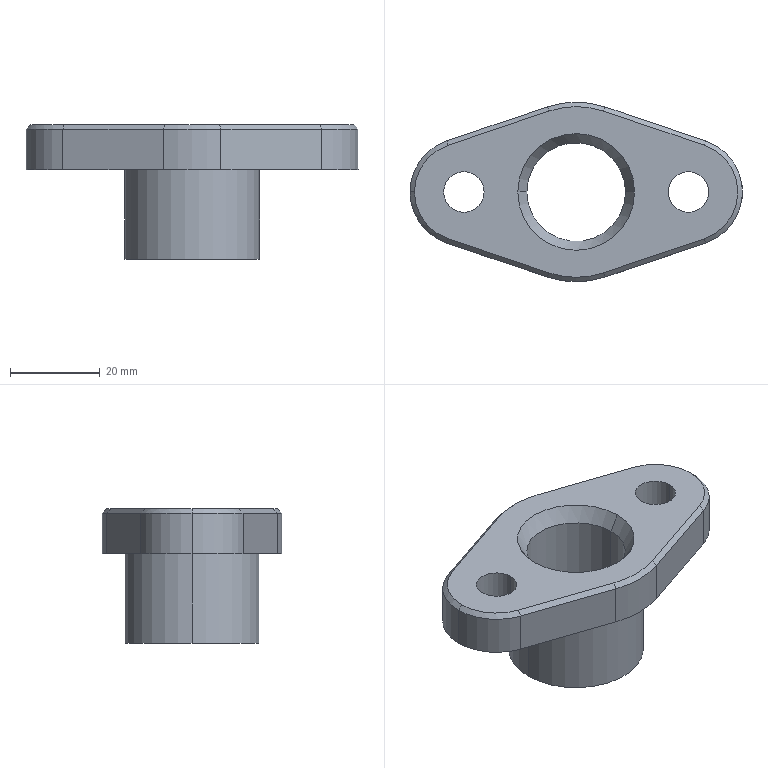Component | SolidWorks | Part4-1 | 1 solid | 33 faces | box 74 x 40 x 30 mm | volume 22214 mm3 | cylinder 13 | plane 11 | cone 9 | commonest cylinder face diameters 9 x4 24 x3 22 x2 30 x2 40 x2
STEP:
#1=CARTESIAN_POINT('',(-4.595,-1.121,8.543));
#2=VERTEX_POINT('',#1);
#3=CARTESIAN_POINT('',(-4.301,-1.532,8.543));
#4=VERTEX_POINT('',#3);
#5=CARTESIAN_POINT('',(-4.162,-1.121,8.543));
#6=DIRECTION('',(0.,0.,1.));
#7=DIRECTION('',(1.,0.,0.));
#8=AXIS2_PLACEMENT_3D('',#5,#6,#7);
#9=CIRCLE('',#8,0.4331);
#10=EDGE_CURVE('',#2,#4,#9,.T.);
#11=ORIENTED_EDGE('',*,*,#10,.F.);
#12=CARTESIAN_POINT('',(-4.635,-1.121,8.504));
#13=VERTEX_POINT('',#12);
#14=CARTESIAN_POINT('',(-4.595,-1.121,8.543));
#15=DIRECTION('',(-0.7071,0.,-0.7071));
#16=VECTOR('',#15,39.37);
#17=LINE('',#14,#16);
#18=EDGE_CURVE('',#2,#13,#17,.T.);
#19=ORIENTED_EDGE('',*,*,#18,.T.);
#20=CARTESIAN_POINT('',(-4.313,-1.569,8.504));
#21=VERTEX_POINT('',#20);
#22=CARTESIAN_POINT('',(-4.162,-1.121,8.504));
#23=DIRECTION('',(0.,0.,-1.));
#24=DIRECTION('',(1.,0.,0.));
#25=AXIS2_PLACEMENT_3D('',#22,#23,#24);
#26=CIRCLE('',#25,0.4724);
#27=EDGE_CURVE('',#21,#13,#26,.T.);
#28=ORIENTED_EDGE('',*,*,#27,.F.);
#29=CARTESIAN_POINT('',(-4.313,-1.569,8.504));
#30=DIRECTION('',(0.2263,0.6699,0.7071));
#31=VECTOR('',#30,39.37);
#32=LINE('',#29,#31);
#33=EDGE_CURVE('',#21,#4,#32,.T.);
#34=ORIENTED_EDGE('',*,*,#33,.T.);
#35=EDGE_LOOP('',(#11,#19,#28,#34));
#36=FACE_OUTER_BOUND('',#35,.T.);
#37=CARTESIAN_POINT('',(-4.162,-1.121,8.543));
#38=DIRECTION('',(0.,0.,-1.));
#39=DIRECTION('',(-1.,0.,0.));
#40=AXIS2_PLACEMENT_3D('',#37,#38,#39);
#41=CONICAL_SURFACE('',#40,0.4331,0.7854);
#42=ADVANCED_FACE('',(#36),#41,.T.);
#43=CARTESIAN_POINT('',(-2.745,-1.121,7.499));
#44=VERTEX_POINT('',#43);
#45=CARTESIAN_POINT('',(-3.611,-1.121,7.499));
#46=VERTEX_POINT('',#45);
#47=CARTESIAN_POINT('',(-3.178,-1.121,7.499));
#48=DIRECTION('',(0.,0.,-1.));
#49=DIRECTION('',(-1.,0.,0.));
#50=AXIS2_PLACEMENT_3D('',#47,#48,#49);
#51=CIRCLE('',#50,0.4331);
#52=EDGE_CURVE('',#44,#46,#51,.T.);
#53=ORIENTED_EDGE('',*,*,#52,.F.);
#54=CARTESIAN_POINT('',(-2.666,-1.121,7.362));
#55=VERTEX_POINT('',#54);
#56=CARTESIAN_POINT('',(-2.745,-1.121,7.499));
#57=DIRECTION('',(0.5,0.,-0.866));
#58=VECTOR('',#57,39.37);
#59=LINE('',#56,#58);
#60=EDGE_CURVE('',#44,#55,#59,.T.);
#61=ORIENTED_EDGE('',*,*,#60,.T.);
#62=CARTESIAN_POINT('',(-3.69,-1.121,7.362));
#63=VERTEX_POINT('',#62);
#64=CARTESIAN_POINT('',(-3.178,-1.121,7.362));
#65=DIRECTION('',(0.,0.,1.));
#66=DIRECTION('',(-1.,0.,0.));
#67=AXIS2_PLACEMENT_3D('',#64,#65,#66);
#68=CIRCLE('',#67,0.5118);
#69=EDGE_CURVE('',#63,#55,#68,.T.);
#70=ORIENTED_EDGE('',*,*,#69,.F.);
#71=CARTESIAN_POINT('',(-3.611,-1.121,7.499));
#72=DIRECTION('',(-0.5,0.,-0.866));
#73=VECTOR('',#72,39.37);
#74=LINE('',#71,#73);
#75=EDGE_CURVE('',#46,#63,#74,.T.);
#76=ORIENTED_EDGE('',*,*,#75,.F.);
#77=EDGE_LOOP('',(#53,#61,#70,#76));
#78=FACE_OUTER_BOUND('',#77,.T.);
#79=CARTESIAN_POINT('',(-3.178,-1.121,7.499));
#80=DIRECTION('',(0.,0.,-1.));
#81=DIRECTION('',(-1.,0.,0.));
#82=AXIS2_PLACEMENT_3D('',#79,#80,#81);
#83=CONICAL_SURFACE('',#82,0.4331,0.5236);
#84=ADVANCED_FACE('',(#78),#83,.F.);
#85=CARTESIAN_POINT('',(-3.611,-1.121,8.407));
#86=VERTEX_POINT('',#85);
#87=CARTESIAN_POINT('',(-2.745,-1.121,8.407));
#88=VERTEX_POINT('',#87);
#89=CARTESIAN_POINT('',(-3.178,-1.121,8.407));
#90=DIRECTION('',(0.,0.,1.));
#91=DIRECTION('',(1.,0.,0.));
#92=AXIS2_PLACEMENT_3D('',#89,#90,#91);
#93=CIRCLE('',#92,0.4331);
#94=EDGE_CURVE('',#86,#88,#93,.T.);
#95=ORIENTED_EDGE('',*,*,#94,.F.);
#96=CARTESIAN_POINT('',(-3.69,-1.121,8.543));
#97=VERTEX_POINT('',#96);
#98=CARTESIAN_POINT('',(-3.611,-1.121,8.407));
#99=DIRECTION('',(-0.5,0.,0.866));
#100=VECTOR('',#99,39.37);
#101=LINE('',#98,#100);
#102=EDGE_CURVE('',#86,#97,#101,.T.);
#103=ORIENTED_EDGE('',*,*,#102,.T.);
#104=CARTESIAN_POINT('',(-2.666,-1.121,8.543));
#105=VERTEX_POINT('',#104);
#106=CARTESIAN_POINT('',(-3.178,-1.121,8.543));
#107=DIRECTION('',(0.,0.,-1.));
#108=DIRECTION('',(1.,0.,0.));
#109=AXIS2_PLACEMENT_3D('',#106,#107,#108);
#110=CIRCLE('',#109,0.5118);
#111=EDGE_CURVE('',#105,#97,#110,.T.);
#112=ORIENTED_EDGE('',*,*,#111,.F.);
#113=CARTESIAN_POINT('',(-2.745,-1.121,8.407));
#114=DIRECTION('',(0.5,0.,0.866));
#115=VECTOR('',#114,39.37);
#116=LINE('',#113,#115);
#117=EDGE_CURVE('',#88,#105,#116,.T.);
#118=ORIENTED_EDGE('',*,*,#117,.F.);
#119=EDGE_LOOP('',(#95,#103,#112,#118));
#120=FACE_OUTER_BOUND('',#119,.T.);
#121=CARTESIAN_POINT('',(-3.178,-1.121,8.407));
#122=DIRECTION('',(0.,0.,1.));
#123=DIRECTION('',(1.,0.,0.));
#124=AXIS2_PLACEMENT_3D('',#121,#122,#123);
#125=CONICAL_SURFACE('',#124,0.4331,0.5236);
#126=ADVANCED_FACE('',(#120),#125,.F.);
#127=ORIENTED_EDGE('',*,*,#52,.T.);
#128=CARTESIAN_POINT('',(-3.611,-1.121,7.362));
#129=DIRECTION('',(0.,0.,1.));
#130=VECTOR('',#129,39.37);
#131=LINE('',#128,#130);
#132=EDGE_CURVE('',#46,#86,#131,.T.);
#133=ORIENTED_EDGE('',*,*,#132,.T.);
#134=ORIENTED_EDGE('',*,*,#94,.T.);
#135=CARTESIAN_POINT('',(-2.745,-1.121,7.362));
#136=DIRECTION('',(0.,0.,1.));
#137=VECTOR('',#136,39.37);
#138=LINE('',#135,#137);
#139=EDGE_CURVE('',#44,#88,#138,.T.);
#140=ORIENTED_EDGE('',*,*,#139,.F.);
#141=EDGE_LOOP('',(#127,#133,#134,#140));
#142=FACE_OUTER_BOUND('',#141,.T.);
#143=CARTESIAN_POINT('',(-3.178,-1.121,7.362));
#144=DIRECTION('',(0.,0.,1.));
#145=DIRECTION('',(1.,0.,0.));
#146=AXIS2_PLACEMENT_3D('',#143,#144,#145);
#147=CYLINDRICAL_SURFACE('',#146,0.4331);
#148=ADVANCED_FACE('',(#142),#147,.F.);
#149=CARTESIAN_POINT('',(-3.768,-1.121,7.362));
#150=VERTEX_POINT('',#149);
#151=CARTESIAN_POINT('',(-2.587,-1.121,7.362));
#152=VERTEX_POINT('',#151);
#153=CARTESIAN_POINT('',(-3.178,-1.121,7.362));
#154=DIRECTION('',(0.,0.,-1.));
#155=DIRECTION('',(-1.,0.,0.));
#156=AXIS2_PLACEMENT_3D('',#153,#154,#155);
#157=CIRCLE('',#156,0.5906);
#158=EDGE_CURVE('',#150,#152,#157,.T.);
#159=ORIENTED_EDGE('',*,*,#158,.F.);
#160=CARTESIAN_POINT('',(-3.768,-1.121,8.15));
#161=VERTEX_POINT('',#160);
#162=CARTESIAN_POINT('',(-3.768,-1.121,7.362));
#163=DIRECTION('',(0.,0.,1.));
#164=VECTOR('',#163,39.37);
#165=LINE('',#162,#164);
#166=EDGE_CURVE('',#150,#161,#165,.T.);
#167=ORIENTED_EDGE('',*,*,#166,.T.);
#168=CARTESIAN_POINT('',(-2.587,-1.121,8.15));
#169=VERTEX_POINT('',#168);
#170=CARTESIAN_POINT('',(-3.178,-1.121,8.15));
#171=DIRECTION('',(0.,0.,-1.));
#172=DIRECTION('',(1.,0.,0.));
#173=AXIS2_PLACEMENT_3D('',#170,#171,#172);
#174=CIRCLE('',#173,0.5906);
#175=EDGE_CURVE('',#161,#169,#174,.T.);
#176=ORIENTED_EDGE('',*,*,#175,.T.);
#177=CARTESIAN_POINT('',(-2.587,-1.121,7.362));
#178=DIRECTION('',(0.,0.,1.));
#179=VECTOR('',#178,39.37);
#180=LINE('',#177,#179);
#181=EDGE_CURVE('',#152,#169,#180,.T.);
#182=ORIENTED_EDGE('',*,*,#181,.F.);
#183=EDGE_LOOP('',(#159,#167,#176,#182));
#184=FACE_OUTER_BOUND('',#183,.T.);
#185=CARTESIAN_POINT('',(-3.178,-1.121,7.362));
#186=DIRECTION('',(0.,0.,1.));
#187=DIRECTION('',(1.,0.,0.));
#188=AXIS2_PLACEMENT_3D('',#185,#186,#187);
#189=CYLINDRICAL_SURFACE('',#188,0.5906);
#190=ADVANCED_FACE('',(#184),#189,.T.);
#191=CARTESIAN_POINT('',(-4.339,-1.121,8.543));
#192=VERTEX_POINT('',#191);
#193=CARTESIAN_POINT('',(-3.985,-1.121,8.543));
#194=VERTEX_POINT('',#193);
#195=CARTESIAN_POINT('',(-4.162,-1.121,8.543));
#196=DIRECTION('',(0.,0.,1.));
#197=DIRECTION('',(1.,0.,0.));
#198=AXIS2_PLACEMENT_3D('',#195,#196,#197);
#199=CIRCLE('',#198,0.1772);
#200=EDGE_CURVE('',#192,#194,#199,.T.);
#201=ORIENTED_EDGE('',*,*,#200,.T.);
#202=CARTESIAN_POINT('',(-3.985,-1.121,8.15));
#203=VERTEX_POINT('',#202);
#204=CARTESIAN_POINT('',(-3.985,-1.121,8.543));
#205=DIRECTION('',(0.,0.,-1.));
#206=VECTOR('',#205,39.37);
#207=LINE('',#204,#206);
#208=EDGE_CURVE('',#194,#203,#207,.T.);
#209=ORIENTED_EDGE('',*,*,#208,.T.);
#210=CARTESIAN_POINT('',(-4.339,-1.121,8.15));
#211=VERTEX_POINT('',#210);
#212=CARTESIAN_POINT('',(-4.162,-1.121,8.15));
#213=DIRECTION('',(0.,0.,1.));
#214=DIRECTION('',(1.,0.,0.));
#215=AXIS2_PLACEMENT_3D('',#212,#213,#214);
#216=CIRCLE('',#215,0.1772);
#217=EDGE_CURVE('',#211,#203,#216,.T.);
#218=ORIENTED_EDGE('',*,*,#217,.F.);
#219=CARTESIAN_POINT('',(-4.339,-1.121,8.543));
#220=DIRECTION('',(0.,0.,-1.));
#221=VECTOR('',#220,39.37);
#222=LINE('',#219,#221);
#223=EDGE_CURVE('',#192,#211,#222,.T.);
#224=ORIENTED_EDGE('',*,*,#223,.F.);
#225=EDGE_LOOP('',(#201,#209,#218,#224));
#226=FACE_OUTER_BOUND('',#225,.T.);
#227=CARTESIAN_POINT('',(-4.162,-1.121,8.543));
#228=DIRECTION('',(0.,0.,-1.));
#229=DIRECTION('',(-1.,0.,0.));
#230=AXIS2_PLACEMENT_3D('',#227,#228,#229);
#231=CYLINDRICAL_SURFACE('',#230,0.1772);
#232=ADVANCED_FACE('',(#226),#231,.F.);
#233=CARTESIAN_POINT('',(-2.371,-1.121,8.543));
#234=VERTEX_POINT('',#233);
#235=CARTESIAN_POINT('',(-2.016,-1.121,8.543));
#236=VERTEX_POINT('',#235);
#237=CARTESIAN_POINT('',(-2.194,-1.121,8.543));
#238=DIRECTION('',(0.,0.,1.));
#239=DIRECTION('',(1.,0.,0.));
#240=AXIS2_PLACEMENT_3D('',#237,#238,#239);
#241=CIRCLE('',#240,0.1772);
#242=EDGE_CURVE('',#234,#236,#241,.T.);
#243=ORIENTED_EDGE('',*,*,#242,.T.);
#244=CARTESIAN_POINT('',(-2.016,-1.121,8.15));
#245=VERTEX_POINT('',#244);
#246=CARTESIAN_POINT('',(-2.016,-1.121,8.543));
#247=DIRECTION('',(0.,0.,-1.));
#248=VECTOR('',#247,39.37);
#249=LINE('',#246,#248);
#250=EDGE_CURVE('',#236,#245,#249,.T.);
#251=ORIENTED_EDGE('',*,*,#250,.T.);
#252=CARTESIAN_POINT('',(-2.371,-1.121,8.15));
#253=VERTEX_POINT('',#252);
#254=CARTESIAN_POINT('',(-2.194,-1.121,8.15));
#255=DIRECTION('',(0.,0.,1.));
#256=DIRECTION('',(1.,0.,0.));
#257=AXIS2_PLACEMENT_3D('',#254,#255,#256);
#258=CIRCLE('',#257,0.1772);
#259=EDGE_CURVE('',#253,#245,#258,.T.);
#260=ORIENTED_EDGE('',*,*,#259,.F.);
#261=CARTESIAN_POINT('',(-2.371,-1.121,8.543));
#262=DIRECTION('',(0.,0.,-1.));
#263=VECTOR('',#262,39.37);
#264=LINE('',#261,#263);
#265=EDGE_CURVE('',#234,#253,#264,.T.);
#266=ORIENTED_EDGE('',*,*,#265,.F.);
#267=EDGE_LOOP('',(#243,#251,#260,#266));
#268=FACE_OUTER_BOUND('',#267,.T.);
#269=CARTESIAN_POINT('',(-2.194,-1.121,8.543));
#270=DIRECTION('',(0.,0.,-1.));
#271=DIRECTION('',(-1.,0.,0.));
#272=AXIS2_PLACEMENT_3D('',#269,#270,#271);
#273=CYLINDRICAL_SURFACE('',#272,0.1772);
#274=ADVANCED_FACE('',(#268),#273,.F.);
#275=ORIENTED_EDGE('',*,*,#27,.T.);
#276=CARTESIAN_POINT('',(-4.635,-1.121,8.15));
#277=VERTEX_POINT('',#276);
#278=CARTESIAN_POINT('',(-4.635,-1.121,8.543));
#279=DIRECTION('',(0.,0.,-1.));
#280=VECTOR('',#279,39.37);
#281=LINE('',#278,#280);
#282=EDGE_CURVE('',#13,#277,#281,.T.);
#283=ORIENTED_EDGE('',*,*,#282,.T.);
#284=CARTESIAN_POINT('',(-4.313,-1.569,8.15));
#285=VERTEX_POINT('',#284);
#286=CARTESIAN_POINT('',(-4.162,-1.121,8.15));
#287=DIRECTION('',(0.,0.,1.));
#288=DIRECTION('',(1.,0.,0.));
#289=AXIS2_PLACEMENT_3D('',#286,#287,#288);
#290=CIRCLE('',#289,0.4724);
#291=EDGE_CURVE('',#277,#285,#290,.T.);
#292=ORIENTED_EDGE('',*,*,#291,.T.);
#293=CARTESIAN_POINT('',(-4.313,-1.569,8.543));
#294=DIRECTION('',(0.,0.,-1.));
#295=VECTOR('',#294,39.37);
#296=LINE('',#293,#295);
#297=EDGE_CURVE('',#21,#285,#296,.T.);
#298=ORIENTED_EDGE('',*,*,#297,.F.);
#299=EDGE_LOOP('',(#275,#283,#292,#298));
#300=FACE_OUTER_BOUND('',#299,.T.);
#301=CARTESIAN_POINT('',(-4.162,-1.121,8.543));
#302=DIRECTION('',(0.,0.,-1.));
#303=DIRECTION('',(-1.,0.,0.));
#304=AXIS2_PLACEMENT_3D('',#301,#302,#303);
#305=CYLINDRICAL_SURFACE('',#304,0.4724);
#306=ADVANCED_FACE('',(#300),#305,.T.);
#307=CARTESIAN_POINT('',(-3.417,-0.4128,8.543));
#308=VERTEX_POINT('',#307);
#309=CARTESIAN_POINT('',(-4.301,-0.7112,8.543));
#310=VERTEX_POINT('',#309);
#311=CARTESIAN_POINT('',(-4.301,-0.7112,8.543));
#312=DIRECTION('',(-0.9474,-0.32,0.));
#313=VECTOR('',#312,39.37);
#314=LINE('',#311,#313);
#315=EDGE_CURVE('',#308,#310,#314,.T.);
#316=ORIENTED_EDGE('',*,*,#315,.T.);
#317=CARTESIAN_POINT('',(-4.162,-1.121,8.543));
#318=DIRECTION('',(0.,0.,1.));
#319=DIRECTION('',(1.,0.,0.));
#320=AXIS2_PLACEMENT_3D('',#317,#318,#319);
#321=CIRCLE('',#320,0.4331);
#322=EDGE_CURVE('',#310,#2,#321,.T.);
#323=ORIENTED_EDGE('',*,*,#322,.T.);
#324=ORIENTED_EDGE('',*,*,#10,.T.);
#325=CARTESIAN_POINT('',(-3.417,-1.83,8.543));
#326=VERTEX_POINT('',#325);
#327=CARTESIAN_POINT('',(-3.417,-1.83,8.543));
#328=DIRECTION('',(0.9474,-0.32,0.));
#329=VECTOR('',#328,39.37);
#330=LINE('',#327,#329);
#331=EDGE_CURVE('',#4,#326,#330,.T.);
#332=ORIENTED_EDGE('',*,*,#331,.T.);
#333=CARTESIAN_POINT('',(-2.939,-1.83,8.543));
#334=VERTEX_POINT('',#333);
#335=CARTESIAN_POINT('',(-3.178,-1.121,8.543));
#336=DIRECTION('',(0.,0.,1.));
#337=DIRECTION('',(1.,0.,0.));
#338=AXIS2_PLACEMENT_3D('',#335,#336,#337);
#339=CIRCLE('',#338,0.748);
#340=EDGE_CURVE('',#326,#334,#339,.T.);
#341=ORIENTED_EDGE('',*,*,#340,.T.);
#342=CARTESIAN_POINT('',(-2.055,-1.532,8.543));
#343=VERTEX_POINT('',#342);
#344=CARTESIAN_POINT('',(-2.055,-1.532,8.543));
#345=DIRECTION('',(0.9474,0.32,0.));
#346=VECTOR('',#345,39.37);
#347=LINE('',#344,#346);
#348=EDGE_CURVE('',#334,#343,#347,.T.);
#349=ORIENTED_EDGE('',*,*,#348,.T.);
#350=CARTESIAN_POINT('',(-2.055,-0.7112,8.543));
#351=VERTEX_POINT('',#350);
#352=CARTESIAN_POINT('',(-2.194,-1.121,8.543));
#353=DIRECTION('',(0.,0.,1.));
#354=DIRECTION('',(1.,0.,0.));
#355=AXIS2_PLACEMENT_3D('',#352,#353,#354);
#356=CIRCLE('',#355,0.4331);
#357=EDGE_CURVE('',#343,#351,#356,.T.);
#358=ORIENTED_EDGE('',*,*,#357,.T.);
#359=CARTESIAN_POINT('',(-2.939,-0.4128,8.543));
#360=VERTEX_POINT('',#359);
#361=CARTESIAN_POINT('',(-2.939,-0.4128,8.543));
#362=DIRECTION('',(-0.9474,0.32,0.));
#363=VECTOR('',#362,39.37);
#364=LINE('',#361,#363);
#365=EDGE_CURVE('',#351,#360,#364,.T.);
#366=ORIENTED_EDGE('',*,*,#365,.T.);
#367=CARTESIAN_POINT('',(-3.178,-1.121,8.543));
#368=DIRECTION('',(0.,0.,1.));
#369=DIRECTION('',(1.,0.,0.));
#370=AXIS2_PLACEMENT_3D('',#367,#368,#369);
#371=CIRCLE('',#370,0.748);
#372=EDGE_CURVE('',#360,#308,#371,.T.);
#373=ORIENTED_EDGE('',*,*,#372,.T.);
#374=EDGE_LOOP('',(#316,#323,#324,#332,#341,#349,#358,#366,#373));
#375=FACE_OUTER_BOUND('',#374,.T.);
#376=ORIENTED_EDGE('',*,*,#111,.T.);
#377=CARTESIAN_POINT('',(-3.178,-1.121,8.543));
#378=DIRECTION('',(0.,0.,-1.));
#379=DIRECTION('',(1.,0.,0.));
#380=AXIS2_PLACEMENT_3D('',#377,#378,#379);
#381=CIRCLE('',#380,0.5118);
#382=EDGE_CURVE('',#97,#105,#381,.T.);
#383=ORIENTED_EDGE('',*,*,#382,.T.);
#384=EDGE_LOOP('',(#376,#383));
#385=FACE_BOUND('',#384,.T.);
#386=ORIENTED_EDGE('',*,*,#242,.F.);
#387=CARTESIAN_POINT('',(-2.194,-1.121,8.543));
#388=DIRECTION('',(0.,0.,1.));
#389=DIRECTION('',(1.,0.,0.));
#390=AXIS2_PLACEMENT_3D('',#387,#388,#389);
#391=CIRCLE('',#390,0.1772);
#392=EDGE_CURVE('',#236,#234,#391,.T.);
#393=ORIENTED_EDGE('',*,*,#392,.F.);
#394=EDGE_LOOP('',(#386,#393));
#395=FACE_BOUND('',#394,.T.);
#396=ORIENTED_EDGE('',*,*,#200,.F.);
#397=CARTESIAN_POINT('',(-4.162,-1.121,8.543));
#398=DIRECTION('',(0.,0.,1.));
#399=DIRECTION('',(1.,0.,0.));
#400=AXIS2_PLACEMENT_3D('',#397,#398,#399);
#401=CIRCLE('',#400,0.1772);
#402=EDGE_CURVE('',#194,#192,#401,.T.);
#403=ORIENTED_EDGE('',*,*,#402,.F.);
#404=EDGE_LOOP('',(#396,#403));
#405=FACE_BOUND('',#404,.T.);
#406=CARTESIAN_POINT('',(-4.162,-1.121,8.543));
#407=DIRECTION('',(0.,0.,1.));
#408=DIRECTION('',(1.,0.,0.));
#409=AXIS2_PLACEMENT_3D('',#406,#407,#408);
#410=PLANE('',#409);
#411=ADVANCED_FACE('',(#375,#385,#395,#405),#410,.T.);
#412=CARTESIAN_POINT('',(-3.178,-1.121,8.15));
#413=DIRECTION('',(0.,0.,-1.));
#414=DIRECTION('',(1.,0.,0.));
#415=AXIS2_PLACEMENT_3D('',#412,#413,#414);
#416=CIRCLE('',#415,0.5906);
#417=EDGE_CURVE('',#169,#161,#416,.T.);
#418=ORIENTED_EDGE('',*,*,#417,.F.);
#419=ORIENTED_EDGE('',*,*,#175,.F.);
#420=EDGE_LOOP('',(#418,#419));
#421=FACE_BOUND('',#420,.T.);
#422=CARTESIAN_POINT('',(-4.313,-0.6739,8.15));
#423=VERTEX_POINT('',#422);
#424=CARTESIAN_POINT('',(-4.162,-1.121,8.15));
#425=DIRECTION('',(0.,0.,1.));
#426=DIRECTION('',(1.,0.,0.));
#427=AXIS2_PLACEMENT_3D('',#424,#425,#426);
#428=CIRCLE('',#427,0.4724);
#429=EDGE_CURVE('',#423,#277,#428,.T.);
#430=ORIENTED_EDGE('',*,*,#429,.F.);
#431=CARTESIAN_POINT('',(-3.43,-0.3755,8.15));
#432=VERTEX_POINT('',#431);
#433=CARTESIAN_POINT('',(-4.313,-0.6739,8.15));
#434=DIRECTION('',(-0.9474,-0.32,0.));
#435=VECTOR('',#434,39.37);
#436=LINE('',#433,#435);
#437=EDGE_CURVE('',#432,#423,#436,.T.);
#438=ORIENTED_EDGE('',*,*,#437,.F.);
#439=CARTESIAN_POINT('',(-2.926,-0.3755,8.15));
#440=VERTEX_POINT('',#439);
#441=CARTESIAN_POINT('',(-3.178,-1.121,8.15));
#442=DIRECTION('',(0.,0.,1.));
#443=DIRECTION('',(1.,0.,0.));
#444=AXIS2_PLACEMENT_3D('',#441,#442,#443);
#445=CIRCLE('',#444,0.7874);
#446=EDGE_CURVE('',#440,#432,#445,.T.);
#447=ORIENTED_EDGE('',*,*,#446,.F.);
#448=CARTESIAN_POINT('',(-2.042,-0.6739,8.15));
#449=VERTEX_POINT('',#448);
#450=CARTESIAN_POINT('',(-2.042,-0.6739,8.15));
#451=DIRECTION('',(-0.9474,0.32,0.));
#452=VECTOR('',#451,39.37);
#453=LINE('',#450,#452);
#454=EDGE_CURVE('',#449,#440,#453,.T.);
#455=ORIENTED_EDGE('',*,*,#454,.F.);
#456=CARTESIAN_POINT('',(-2.042,-1.569,8.15));
#457=VERTEX_POINT('',#456);
#458=CARTESIAN_POINT('',(-2.194,-1.121,8.15));
#459=DIRECTION('',(0.,0.,1.));
#460=DIRECTION('',(-1.,0.,0.));
#461=AXIS2_PLACEMENT_3D('',#458,#459,#460);
#462=CIRCLE('',#461,0.4724);
#463=EDGE_CURVE('',#457,#449,#462,.T.);
#464=ORIENTED_EDGE('',*,*,#463,.F.);
#465=CARTESIAN_POINT('',(-2.926,-1.867,8.15));
#466=VERTEX_POINT('',#465);
#467=CARTESIAN_POINT('',(-2.042,-1.569,8.15));
#468=DIRECTION('',(0.9474,0.32,0.));
#469=VECTOR('',#468,39.37);
#470=LINE('',#467,#469);
#471=EDGE_CURVE('',#466,#457,#470,.T.);
#472=ORIENTED_EDGE('',*,*,#471,.F.);
#473=CARTESIAN_POINT('',(-3.43,-1.867,8.15));
#474=VERTEX_POINT('',#473);
#475=CARTESIAN_POINT('',(-3.178,-1.121,8.15));
#476=DIRECTION('',(0.,0.,1.));
#477=DIRECTION('',(1.,0.,0.));
#478=AXIS2_PLACEMENT_3D('',#475,#476,#477);
#479=CIRCLE('',#478,0.7874);
#480=EDGE_CURVE('',#474,#466,#479,.T.);
#481=ORIENTED_EDGE('',*,*,#480,.F.);
#482=CARTESIAN_POINT('',(-4.313,-1.569,8.15));
#483=DIRECTION('',(0.9474,-0.32,0.));
#484=VECTOR('',#483,39.37);
#485=LINE('',#482,#484);
#486=EDGE_CURVE('',#285,#474,#485,.T.);
#487=ORIENTED_EDGE('',*,*,#486,.F.);
#488=ORIENTED_EDGE('',*,*,#291,.F.);
#489=EDGE_LOOP('',(#430,#438,#447,#455,#464,#472,#481,#487,#488));
#490=FACE_OUTER_BOUND('',#489,.T.);
#491=ORIENTED_EDGE('',*,*,#259,.T.);
#492=CARTESIAN_POINT('',(-2.194,-1.121,8.15));
#493=DIRECTION('',(0.,0.,1.));
#494=DIRECTION('',(1.,0.,0.));
#495=AXIS2_PLACEMENT_3D('',#492,#493,#494);
#496=CIRCLE('',#495,0.1772);
#497=EDGE_CURVE('',#245,#253,#496,.T.);
#498=ORIENTED_EDGE('',*,*,#497,.T.);
#499=EDGE_LOOP('',(#491,#498));
#500=FACE_BOUND('',#499,.T.);
#501=ORIENTED_EDGE('',*,*,#217,.T.);
#502=CARTESIAN_POINT('',(-4.162,-1.121,8.15));
#503=DIRECTION('',(0.,0.,1.));
#504=DIRECTION('',(1.,0.,0.));
#505=AXIS2_PLACEMENT_3D('',#502,#503,#504);
#506=CIRCLE('',#505,0.1772);
#507=EDGE_CURVE('',#203,#211,#506,.T.);
#508=ORIENTED_EDGE('',*,*,#507,.T.);
#509=EDGE_LOOP('',(#501,#508));
#510=FACE_BOUND('',#509,.T.);
#511=CARTESIAN_POINT('',(-4.162,-1.121,8.15));
#512=DIRECTION('',(0.,0.,1.));
#513=DIRECTION('',(1.,0.,0.));
#514=AXIS2_PLACEMENT_3D('',#511,#512,#513);
#515=PLANE('',#514);
#516=ADVANCED_FACE('',(#421,#490,#500,#510),#515,.F.);
#517=ORIENTED_EDGE('',*,*,#282,.F.);
#518=CARTESIAN_POINT('',(-4.313,-0.6739,8.504));
#519=VERTEX_POINT('',#518);
#520=CARTESIAN_POINT('',(-4.162,-1.121,8.504));
#521=DIRECTION('',(0.,0.,-1.));
#522=DIRECTION('',(1.,0.,0.));
#523=AXIS2_PLACEMENT_3D('',#520,#521,#522);
#524=CIRCLE('',#523,0.4724);
#525=EDGE_CURVE('',#13,#519,#524,.T.);
#526=ORIENTED_EDGE('',*,*,#525,.T.);
#527=CARTESIAN_POINT('',(-4.313,-0.6739,8.543));
#528=DIRECTION('',(0.,0.,-1.));
#529=VECTOR('',#528,39.37);
#530=LINE('',#527,#529);
#531=EDGE_CURVE('',#519,#423,#530,.T.);
#532=ORIENTED_EDGE('',*,*,#531,.T.);
#533=ORIENTED_EDGE('',*,*,#429,.T.);
#534=EDGE_LOOP('',(#517,#526,#532,#533));
#535=FACE_OUTER_BOUND('',#534,.T.);
#536=CARTESIAN_POINT('',(-4.162,-1.121,8.543));
#537=DIRECTION('',(0.,0.,-1.));
#538=DIRECTION('',(-1.,0.,0.));
#539=AXIS2_PLACEMENT_3D('',#536,#537,#538);
#540=CYLINDRICAL_SURFACE('',#539,0.4724);
#541=ADVANCED_FACE('',(#535),#540,.T.);
#542=CARTESIAN_POINT('',(-3.43,-1.867,8.504));
#543=VERTEX_POINT('',#542);
#544=CARTESIAN_POINT('',(-3.43,-1.867,8.543));
#545=DIRECTION('',(0.,0.,-1.));
#546=VECTOR('',#545,39.37);
#547=LINE('',#544,#546);
#548=EDGE_CURVE('',#543,#474,#547,.T.);
#549=ORIENTED_EDGE('',*,*,#548,.F.);
#550=CARTESIAN_POINT('',(-4.313,-1.569,8.504));
#551=DIRECTION('',(-0.9474,0.32,0.));
#552=VECTOR('',#551,39.37);
#553=LINE('',#550,#552);
#554=EDGE_CURVE('',#543,#21,#553,.T.);
#555=ORIENTED_EDGE('',*,*,#554,.T.);
#556=ORIENTED_EDGE('',*,*,#297,.T.);
#557=ORIENTED_EDGE('',*,*,#486,.T.);
#558=EDGE_LOOP('',(#549,#555,#556,#557));
#559=FACE_OUTER_BOUND('',#558,.T.);
#560=CARTESIAN_POINT('',(-4.313,-1.569,8.543));
#561=DIRECTION('',(0.32,0.9474,0.));
#562=DIRECTION('',(-0.9474,0.32,0.));
#563=AXIS2_PLACEMENT_3D('',#560,#561,#562);
#564=PLANE('',#563);
#565=ADVANCED_FACE('',(#559),#564,.F.);
#566=CARTESIAN_POINT('',(-2.926,-1.867,8.504));
#567=VERTEX_POINT('',#566);
#568=CARTESIAN_POINT('',(-2.926,-1.867,8.543));
#569=DIRECTION('',(0.,0.,-1.));
#570=VECTOR('',#569,39.37);
#571=LINE('',#568,#570);
#572=EDGE_CURVE('',#567,#466,#571,.T.);
#573=ORIENTED_EDGE('',*,*,#572,.F.);
#574=CARTESIAN_POINT('',(-3.178,-1.121,8.504));
#575=DIRECTION('',(0.,0.,-1.));
#576=DIRECTION('',(1.,0.,0.));
#577=AXIS2_PLACEMENT_3D('',#574,#575,#576);
#578=CIRCLE('',#577,0.7874);
#579=EDGE_CURVE('',#567,#543,#578,.T.);
#580=ORIENTED_EDGE('',*,*,#579,.T.);
#581=ORIENTED_EDGE('',*,*,#548,.T.);
#582=ORIENTED_EDGE('',*,*,#480,.T.);
#583=EDGE_LOOP('',(#573,#580,#581,#582));
#584=FACE_OUTER_BOUND('',#583,.T.);
#585=CARTESIAN_POINT('',(-3.178,-1.121,8.543));
#586=DIRECTION('',(0.,0.,-1.));
#587=DIRECTION('',(-1.,0.,0.));
#588=AXIS2_PLACEMENT_3D('',#585,#586,#587);
#589=CYLINDRICAL_SURFACE('',#588,0.7874);
#590=ADVANCED_FACE('',(#584),#589,.T.);
#591=CARTESIAN_POINT('',(-2.042,-1.569,8.504));
#592=VERTEX_POINT('',#591);
#593=CARTESIAN_POINT('',(-2.042,-1.569,8.543));
#594=DIRECTION('',(0.,0.,-1.));
#595=VECTOR('',#594,39.37);
#596=LINE('',#593,#595);
#597=EDGE_CURVE('',#592,#457,#596,.T.);
#598=ORIENTED_EDGE('',*,*,#597,.F.);
#599=CARTESIAN_POINT('',(-2.926,-1.867,8.504));
#600=DIRECTION('',(-0.9474,-0.32,0.));
#601=VECTOR('',#600,39.37);
#602=LINE('',#599,#601);
#603=EDGE_CURVE('',#592,#567,#602,.T.);
#604=ORIENTED_EDGE('',*,*,#603,.T.);
#605=ORIENTED_EDGE('',*,*,#572,.T.);
#606=ORIENTED_EDGE('',*,*,#471,.T.);
#607=EDGE_LOOP('',(#598,#604,#605,#606));
#608=FACE_OUTER_BOUND('',#607,.T.);
#609=CARTESIAN_POINT('',(-2.042,-1.569,8.543));
#610=DIRECTION('',(-0.32,0.9474,0.));
#611=DIRECTION('',(-0.9474,-0.32,0.));
#612=AXIS2_PLACEMENT_3D('',#609,#610,#611);
#613=PLANE('',#612);
#614=ADVANCED_FACE('',(#608),#613,.F.);
#615=CARTESIAN_POINT('',(-2.042,-0.6739,8.504));
#616=VERTEX_POINT('',#615);
#617=CARTESIAN_POINT('',(-2.042,-0.6739,8.543));
#618=DIRECTION('',(0.,0.,-1.));
#619=VECTOR('',#618,39.37);
#620=LINE('',#617,#619);
#621=EDGE_CURVE('',#616,#449,#620,.T.);
#622=ORIENTED_EDGE('',*,*,#621,.F.);
#623=CARTESIAN_POINT('',(-2.194,-1.121,8.504));
#624=DIRECTION('',(0.,0.,-1.));
#625=DIRECTION('',(1.,0.,0.));
#626=AXIS2_PLACEMENT_3D('',#623,#624,#625);
#627=CIRCLE('',#626,0.4724);
#628=EDGE_CURVE('',#616,#592,#627,.T.);
#629=ORIENTED_EDGE('',*,*,#628,.T.);
#630=ORIENTED_EDGE('',*,*,#597,.T.);
#631=ORIENTED_EDGE('',*,*,#463,.T.);
#632=EDGE_LOOP('',(#622,#629,#630,#631));
#633=FACE_OUTER_BOUND('',#632,.T.);
#634=CARTESIAN_POINT('',(-2.194,-1.121,8.543));
#635=DIRECTION('',(0.,0.,-1.));
#636=DIRECTION('',(-1.,0.,0.));
#637=AXIS2_PLACEMENT_3D('',#634,#635,#636);
#638=CYLINDRICAL_SURFACE('',#637,0.4724);
#639=ADVANCED_FACE('',(#633),#638,.T.);
#640=CARTESIAN_POINT('',(-2.926,-0.3755,8.504));
#641=VERTEX_POINT('',#640);
#642=CARTESIAN_POINT('',(-2.926,-0.3755,8.543));
#643=DIRECTION('',(0.,0.,-1.));
#644=VECTOR('',#643,39.37);
#645=LINE('',#642,#644);
#646=EDGE_CURVE('',#641,#440,#645,.T.);
#647=ORIENTED_EDGE('',*,*,#646,.F.);
#648=CARTESIAN_POINT('',(-2.042,-0.6739,8.504));
#649=DIRECTION('',(0.9474,-0.32,0.));
#650=VECTOR('',#649,39.37);
#651=LINE('',#648,#650);
#652=EDGE_CURVE('',#641,#616,#651,.T.);
#653=ORIENTED_EDGE('',*,*,#652,.T.);
#654=ORIENTED_EDGE('',*,*,#621,.T.);
#655=ORIENTED_EDGE('',*,*,#454,.T.);
#656=EDGE_LOOP('',(#647,#653,#654,#655));
#657=FACE_OUTER_BOUND('',#656,.T.);
#658=CARTESIAN_POINT('',(-2.042,-0.6739,8.543));
#659=DIRECTION('',(-0.32,-0.9474,0.));
#660=DIRECTION('',(0.9474,-0.32,0.));
#661=AXIS2_PLACEMENT_3D('',#658,#659,#660);
#662=PLANE('',#661);
#663=ADVANCED_FACE('',(#657),#662,.F.);
#664=CARTESIAN_POINT('',(-3.43,-0.3755,8.504));
#665=VERTEX_POINT('',#664);
#666=CARTESIAN_POINT('',(-3.43,-0.3755,8.543));
#667=DIRECTION('',(0.,0.,-1.));
#668=VECTOR('',#667,39.37);
#669=LINE('',#666,#668);
#670=EDGE_CURVE('',#665,#432,#669,.T.);
#671=ORIENTED_EDGE('',*,*,#670,.F.);
#672=CARTESIAN_POINT('',(-3.178,-1.121,8.504));
#673=DIRECTION('',(0.,0.,-1.));
#674=DIRECTION('',(1.,0.,0.));
#675=AXIS2_PLACEMENT_3D('',#672,#673,#674);
#676=CIRCLE('',#675,0.7874);
#677=EDGE_CURVE('',#665,#641,#676,.T.);
#678=ORIENTED_EDGE('',*,*,#677,.T.);
#679=ORIENTED_EDGE('',*,*,#646,.T.);
#680=ORIENTED_EDGE('',*,*,#446,.T.);
#681=EDGE_LOOP('',(#671,#678,#679,#680));
#682=FACE_OUTER_BOUND('',#681,.T.);
#683=CARTESIAN_POINT('',(-3.178,-1.121,8.543));
#684=DIRECTION('',(0.,0.,-1.));
#685=DIRECTION('',(-1.,0.,0.));
#686=AXIS2_PLACEMENT_3D('',#683,#684,#685);
#687=CYLINDRICAL_SURFACE('',#686,0.7874);
#688=ADVANCED_FACE('',(#682),#687,.T.);
#689=ORIENTED_EDGE('',*,*,#531,.F.);
#690=CARTESIAN_POINT('',(-3.43,-0.3755,8.504));
#691=DIRECTION('',(0.9474,0.32,0.));
#692=VECTOR('',#691,39.37);
#693=LINE('',#690,#692);
#694=EDGE_CURVE('',#519,#665,#693,.T.);
#695=ORIENTED_EDGE('',*,*,#694,.T.);
#696=ORIENTED_EDGE('',*,*,#670,.T.);
#697=ORIENTED_EDGE('',*,*,#437,.T.);
#698=EDGE_LOOP('',(#689,#695,#696,#697));
#699=FACE_OUTER_BOUND('',#698,.T.);
#700=CARTESIAN_POINT('',(-4.313,-0.6739,8.543));
#701=DIRECTION('',(0.32,-0.9474,0.));
#702=DIRECTION('',(0.9474,0.32,0.));
#703=AXIS2_PLACEMENT_3D('',#700,#701,#702);
#704=PLANE('',#703);
#705=ADVANCED_FACE('',(#699),#704,.F.);
#706=ORIENTED_EDGE('',*,*,#250,.F.);
#707=ORIENTED_EDGE('',*,*,#392,.T.);
#708=ORIENTED_EDGE('',*,*,#265,.T.);
#709=ORIENTED_EDGE('',*,*,#497,.F.);
#710=EDGE_LOOP('',(#706,#707,#708,#709));
#711=FACE_OUTER_BOUND('',#710,.T.);
#712=CARTESIAN_POINT('',(-2.194,-1.121,8.543));
#713=DIRECTION('',(0.,0.,-1.));
#714=DIRECTION('',(-1.,0.,0.));
#715=AXIS2_PLACEMENT_3D('',#712,#713,#714);
#716=CYLINDRICAL_SURFACE('',#715,0.1772);
#717=ADVANCED_FACE('',(#711),#716,.F.);
#718=ORIENTED_EDGE('',*,*,#208,.F.);
#719=ORIENTED_EDGE('',*,*,#402,.T.);
#720=ORIENTED_EDGE('',*,*,#223,.T.);
#721=ORIENTED_EDGE('',*,*,#507,.F.);
#722=EDGE_LOOP('',(#718,#719,#720,#721));
#723=FACE_OUTER_BOUND('',#722,.T.);
#724=CARTESIAN_POINT('',(-4.162,-1.121,8.543));
#725=DIRECTION('',(0.,0.,-1.));
#726=DIRECTION('',(-1.,0.,0.));
#727=AXIS2_PLACEMENT_3D('',#724,#725,#726);
#728=CYLINDRICAL_SURFACE('',#727,0.1772);
#729=ADVANCED_FACE('',(#723),#728,.F.);
#730=ORIENTED_EDGE('',*,*,#69,.T.);
#731=CARTESIAN_POINT('',(-3.178,-1.121,7.362));
#732=DIRECTION('',(0.,0.,1.));
#733=DIRECTION('',(-1.,0.,0.));
#734=AXIS2_PLACEMENT_3D('',#731,#732,#733);
#735=CIRCLE('',#734,0.5118);
#736=EDGE_CURVE('',#55,#63,#735,.T.);
#737=ORIENTED_EDGE('',*,*,#736,.T.);
#738=EDGE_LOOP('',(#730,#737));
#739=FACE_BOUND('',#738,.T.);
#740=CARTESIAN_POINT('',(-3.178,-1.121,7.362));
#741=DIRECTION('',(0.,0.,-1.));
#742=DIRECTION('',(-1.,0.,0.));
#743=AXIS2_PLACEMENT_3D('',#740,#741,#742);
#744=CIRCLE('',#743,0.5906);
#745=EDGE_CURVE('',#152,#150,#744,.T.);
#746=ORIENTED_EDGE('',*,*,#745,.T.);
#747=ORIENTED_EDGE('',*,*,#158,.T.);
#748=EDGE_LOOP('',(#746,#747));
#749=FACE_OUTER_BOUND('',#748,.T.);
#750=CARTESIAN_POINT('',(-3.178,-1.121,7.362));
#751=DIRECTION('',(0.,0.,-1.));
#752=DIRECTION('',(-1.,0.,0.));
#753=AXIS2_PLACEMENT_3D('',#750,#751,#752);
#754=PLANE('',#753);
#755=ADVANCED_FACE('',(#739,#749),#754,.T.);
#756=ORIENTED_EDGE('',*,*,#166,.F.);
#757=ORIENTED_EDGE('',*,*,#745,.F.);
#758=ORIENTED_EDGE('',*,*,#181,.T.);
#759=ORIENTED_EDGE('',*,*,#417,.T.);
#760=EDGE_LOOP('',(#756,#757,#758,#759));
#761=FACE_OUTER_BOUND('',#760,.T.);
#762=CARTESIAN_POINT('',(-3.178,-1.121,7.362));
#763=DIRECTION('',(0.,0.,1.));
#764=DIRECTION('',(1.,0.,0.));
#765=AXIS2_PLACEMENT_3D('',#762,#763,#764);
#766=CYLINDRICAL_SURFACE('',#765,0.5906);
#767=ADVANCED_FACE('',(#761),#766,.T.);
#768=ORIENTED_EDGE('',*,*,#132,.F.);
#769=CARTESIAN_POINT('',(-3.178,-1.121,7.499));
#770=DIRECTION('',(0.,0.,-1.));
#771=DIRECTION('',(-1.,0.,0.));
#772=AXIS2_PLACEMENT_3D('',#769,#770,#771);
#773=CIRCLE('',#772,0.4331);
#774=EDGE_CURVE('',#46,#44,#773,.T.);
#775=ORIENTED_EDGE('',*,*,#774,.T.);
#776=ORIENTED_EDGE('',*,*,#139,.T.);
#777=CARTESIAN_POINT('',(-3.178,-1.121,8.407));
#778=DIRECTION('',(0.,0.,1.));
#779=DIRECTION('',(1.,0.,0.));
#780=AXIS2_PLACEMENT_3D('',#777,#778,#779);
#781=CIRCLE('',#780,0.4331);
#782=EDGE_CURVE('',#88,#86,#781,.T.);
#783=ORIENTED_EDGE('',*,*,#782,.T.);
#784=EDGE_LOOP('',(#768,#775,#776,#783));
#785=FACE_OUTER_BOUND('',#784,.T.);
#786=CARTESIAN_POINT('',(-3.178,-1.121,7.362));
#787=DIRECTION('',(0.,0.,1.));
#788=DIRECTION('',(1.,0.,0.));
#789=AXIS2_PLACEMENT_3D('',#786,#787,#788);
#790=CYLINDRICAL_SURFACE('',#789,0.4331);
#791=ADVANCED_FACE('',(#785),#790,.F.);
#792=ORIENTED_EDGE('',*,*,#102,.F.);
#793=ORIENTED_EDGE('',*,*,#782,.F.);
#794=ORIENTED_EDGE('',*,*,#117,.T.);
#795=ORIENTED_EDGE('',*,*,#382,.F.);
#796=EDGE_LOOP('',(#792,#793,#794,#795));
#797=FACE_OUTER_BOUND('',#796,.T.);
#798=CARTESIAN_POINT('',(-3.178,-1.121,8.407));
#799=DIRECTION('',(0.,0.,1.));
#800=DIRECTION('',(1.,0.,0.));
#801=AXIS2_PLACEMENT_3D('',#798,#799,#800);
#802=CONICAL_SURFACE('',#801,0.4331,0.5236);
#803=ADVANCED_FACE('',(#797),#802,.F.);
#804=ORIENTED_EDGE('',*,*,#60,.F.);
#805=ORIENTED_EDGE('',*,*,#774,.F.);
#806=ORIENTED_EDGE('',*,*,#75,.T.);
#807=ORIENTED_EDGE('',*,*,#736,.F.);
#808=EDGE_LOOP('',(#804,#805,#806,#807));
#809=FACE_OUTER_BOUND('',#808,.T.);
#810=CARTESIAN_POINT('',(-3.178,-1.121,7.499));
#811=DIRECTION('',(0.,0.,-1.));
#812=DIRECTION('',(-1.,0.,0.));
#813=AXIS2_PLACEMENT_3D('',#810,#811,#812);
#814=CONICAL_SURFACE('',#813,0.4331,0.5236);
#815=ADVANCED_FACE('',(#809),#814,.F.);
#816=CARTESIAN_POINT('',(-2.042,-1.569,8.504));
#817=DIRECTION('',(-0.2263,0.6699,0.7071));
#818=VECTOR('',#817,39.37);
#819=LINE('',#816,#818);
#820=EDGE_CURVE('',#592,#343,#819,.T.);
#821=ORIENTED_EDGE('',*,*,#820,.F.);
#822=ORIENTED_EDGE('',*,*,#628,.F.);
#823=CARTESIAN_POINT('',(-2.055,-0.7112,8.543));
#824=DIRECTION('',(0.2263,0.6699,-0.7071));
#825=VECTOR('',#824,39.37);
#826=LINE('',#823,#825);
#827=EDGE_CURVE('',#351,#616,#826,.T.);
#828=ORIENTED_EDGE('',*,*,#827,.F.);
#829=ORIENTED_EDGE('',*,*,#357,.F.);
#830=EDGE_LOOP('',(#821,#822,#828,#829));
#831=FACE_OUTER_BOUND('',#830,.T.);
#832=CARTESIAN_POINT('',(-2.194,-1.121,8.543));
#833=DIRECTION('',(0.,0.,-1.));
#834=DIRECTION('',(-1.,0.,0.));
#835=AXIS2_PLACEMENT_3D('',#832,#833,#834);
#836=CONICAL_SURFACE('',#835,0.4331,0.7854);
#837=ADVANCED_FACE('',(#831),#836,.T.);
#838=ORIENTED_EDGE('',*,*,#827,.T.);
#839=ORIENTED_EDGE('',*,*,#652,.F.);
#840=CARTESIAN_POINT('',(-2.939,-0.4128,8.543));
#841=DIRECTION('',(0.2263,0.6699,-0.7071));
#842=VECTOR('',#841,39.37);
#843=LINE('',#840,#842);
#844=EDGE_CURVE('',#360,#641,#843,.T.);
#845=ORIENTED_EDGE('',*,*,#844,.F.);
#846=ORIENTED_EDGE('',*,*,#365,.F.);
#847=EDGE_LOOP('',(#838,#839,#845,#846));
#848=FACE_OUTER_BOUND('',#847,.T.);
#849=CARTESIAN_POINT('',(-3.822,-0.1144,8.543));
#850=DIRECTION('',(0.2263,0.6699,0.7071));
#851=DIRECTION('',(0.9474,-0.32,0.));
#852=AXIS2_PLACEMENT_3D('',#849,#850,#851);
#853=PLANE('',#852);
#854=ADVANCED_FACE('',(#848),#853,.T.);
#855=ORIENTED_EDGE('',*,*,#820,.T.);
#856=ORIENTED_EDGE('',*,*,#348,.F.);
#857=CARTESIAN_POINT('',(-2.926,-1.867,8.504));
#858=DIRECTION('',(-0.2263,0.6699,0.7071));
#859=VECTOR('',#858,39.37);
#860=LINE('',#857,#859);
#861=EDGE_CURVE('',#567,#334,#860,.T.);
#862=ORIENTED_EDGE('',*,*,#861,.F.);
#863=ORIENTED_EDGE('',*,*,#603,.F.);
#864=EDGE_LOOP('',(#855,#856,#862,#863));
#865=FACE_OUTER_BOUND('',#864,.T.);
#866=CARTESIAN_POINT('',(-3.822,-2.129,8.543));
#867=DIRECTION('',(0.2263,-0.6699,0.7071));
#868=DIRECTION('',(-0.9474,-0.32,0.));
#869=AXIS2_PLACEMENT_3D('',#866,#867,#868);
#870=PLANE('',#869);
#871=ADVANCED_FACE('',(#865),#870,.T.);
#872=ORIENTED_EDGE('',*,*,#844,.T.);
#873=ORIENTED_EDGE('',*,*,#677,.F.);
#874=CARTESIAN_POINT('',(-3.417,-0.4128,8.543));
#875=DIRECTION('',(-0.2263,0.6699,-0.7071));
#876=VECTOR('',#875,39.37);
#877=LINE('',#874,#876);
#878=EDGE_CURVE('',#308,#665,#877,.T.);
#879=ORIENTED_EDGE('',*,*,#878,.F.);
#880=ORIENTED_EDGE('',*,*,#372,.F.);
#881=EDGE_LOOP('',(#872,#873,#879,#880));
#882=FACE_OUTER_BOUND('',#881,.T.);
#883=CARTESIAN_POINT('',(-3.178,-1.121,8.543));
#884=DIRECTION('',(0.,0.,-1.));
#885=DIRECTION('',(-1.,0.,0.));
#886=AXIS2_PLACEMENT_3D('',#883,#884,#885);
#887=CONICAL_SURFACE('',#886,0.748,0.7854);
#888=ADVANCED_FACE('',(#882),#887,.T.);
#889=ORIENTED_EDGE('',*,*,#861,.T.);
#890=ORIENTED_EDGE('',*,*,#340,.F.);
#891=CARTESIAN_POINT('',(-3.43,-1.867,8.504));
#892=DIRECTION('',(0.2263,0.6699,0.7071));
#893=VECTOR('',#892,39.37);
#894=LINE('',#891,#893);
#895=EDGE_CURVE('',#543,#326,#894,.T.);
#896=ORIENTED_EDGE('',*,*,#895,.F.);
#897=ORIENTED_EDGE('',*,*,#579,.F.);
#898=EDGE_LOOP('',(#889,#890,#896,#897));
#899=FACE_OUTER_BOUND('',#898,.T.);
#900=CARTESIAN_POINT('',(-3.178,-1.121,8.543));
#901=DIRECTION('',(0.,0.,-1.));
#902=DIRECTION('',(-1.,0.,0.));
#903=AXIS2_PLACEMENT_3D('',#900,#901,#902);
#904=CONICAL_SURFACE('',#903,0.748,0.7854);
#905=ADVANCED_FACE('',(#899),#904,.T.);
#906=ORIENTED_EDGE('',*,*,#878,.T.);
#907=ORIENTED_EDGE('',*,*,#694,.F.);
#908=CARTESIAN_POINT('',(-4.301,-0.7112,8.543));
#909=DIRECTION('',(-0.2263,0.6699,-0.7071));
#910=VECTOR('',#909,39.37);
#911=LINE('',#908,#910);
#912=EDGE_CURVE('',#310,#519,#911,.T.);
#913=ORIENTED_EDGE('',*,*,#912,.F.);
#914=ORIENTED_EDGE('',*,*,#315,.F.);
#915=EDGE_LOOP('',(#906,#907,#913,#914));
#916=FACE_OUTER_BOUND('',#915,.T.);
#917=CARTESIAN_POINT('',(-4.301,-0.7112,8.543));
#918=DIRECTION('',(-0.2263,0.6699,0.7071));
#919=DIRECTION('',(0.9474,0.32,0.));
#920=AXIS2_PLACEMENT_3D('',#917,#918,#919);
#921=PLANE('',#920);
#922=ADVANCED_FACE('',(#916),#921,.T.);
#923=ORIENTED_EDGE('',*,*,#895,.T.);
#924=ORIENTED_EDGE('',*,*,#331,.F.);
#925=ORIENTED_EDGE('',*,*,#33,.F.);
#926=ORIENTED_EDGE('',*,*,#554,.F.);
#927=EDGE_LOOP('',(#923,#924,#925,#926));
#928=FACE_OUTER_BOUND('',#927,.T.);
#929=CARTESIAN_POINT('',(-4.301,-1.532,8.543));
#930=DIRECTION('',(-0.2263,-0.6699,0.7071));
#931=DIRECTION('',(-0.9474,0.32,0.));
#932=AXIS2_PLACEMENT_3D('',#929,#930,#931);
#933=PLANE('',#932);
#934=ADVANCED_FACE('',(#928),#933,.T.);
#935=ORIENTED_EDGE('',*,*,#18,.F.);
#936=ORIENTED_EDGE('',*,*,#322,.F.);
#937=ORIENTED_EDGE('',*,*,#912,.T.);
#938=ORIENTED_EDGE('',*,*,#525,.F.);
#939=EDGE_LOOP('',(#935,#936,#937,#938));
#940=FACE_OUTER_BOUND('',#939,.T.);
#941=CARTESIAN_POINT('',(-4.162,-1.121,8.543));
#942=DIRECTION('',(0.,0.,-1.));
#943=DIRECTION('',(-1.,0.,0.));
#944=AXIS2_PLACEMENT_3D('',#941,#942,#943);
#945=CONICAL_SURFACE('',#944,0.4331,0.7854);
#946=ADVANCED_FACE('',(#940),#945,.T.);
#947=CLOSED_SHELL('',(#42,#84,#126,#148,#190,#232,#274,#306,#411,#516,#541,#565,#590,#614,#639,#663,#688,#705,#717,#729,#755,#767,#791,#803,#815,#837,#854,#871,#888,#905,#922,#934,#946));
#948=MANIFOLD_SOLID_BREP('',#947);
#949=CARTESIAN_POINT('',(0.,0.,0.));
#950=DIRECTION('',(0.,0.,1.));
#951=DIRECTION('',(1.,0.,0.));
#952=AXIS2_PLACEMENT_3D('',#949,#950,#951);
#953=(LENGTH_UNIT()NAMED_UNIT(*)SI_UNIT($,.METRE.));
#954=LENGTH_MEASURE_WITH_UNIT(LENGTH_MEASURE(0.0254),#953);
#955=DIMENSIONAL_EXPONENTS(1.,0.,0.,0.,0.,0.,0.);
#956=(CONVERSION_BASED_UNIT('',#954)LENGTH_UNIT()NAMED_UNIT(#955));
#957=UNCERTAINTY_MEASURE_WITH_UNIT(LENGTH_MEASURE(0.00001),#956,'','');
#958=(NAMED_UNIT(*)PLANE_ANGLE_UNIT()SI_UNIT($,.RADIAN.));
#959=(NAMED_UNIT(*)SI_UNIT($,.STERADIAN.)SOLID_ANGLE_UNIT());
#960=(GEOMETRIC_REPRESENTATION_CONTEXT(3)GLOBAL_UNCERTAINTY_ASSIGNED_CONTEXT((#957))GLOBAL_UNIT_ASSIGNED_CONTEXT((#956,#958,#959))REPRESENTATION_CONTEXT('',''));
#961=ADVANCED_BREP_SHAPE_REPRESENTATION('',(#948,#952),#960);
#962=COLOUR_RGB('',0.7922,0.8196,0.9333);
#963=FILL_AREA_STYLE_COLOUR('',#962);
#964=FILL_AREA_STYLE('',(#963));
#965=SURFACE_STYLE_FILL_AREA(#964);
#966=SURFACE_SIDE_STYLE('',(#965));
#967=SURFACE_STYLE_USAGE(.BOTH.,#966);
#968=PRESENTATION_STYLE_ASSIGNMENT((#967));
#969=STYLED_ITEM('',(#968),#948);
#970=PRESENTATION_LAYER_ASSIGNMENT('','',(#969));
#971=(LENGTH_UNIT()NAMED_UNIT(*)SI_UNIT($,.METRE.));
#972=LENGTH_MEASURE_WITH_UNIT(LENGTH_MEASURE(0.0254),#971);
#973=DIMENSIONAL_EXPONENTS(1.,0.,0.,0.,0.,0.,0.);
#974=(CONVERSION_BASED_UNIT('',#972)LENGTH_UNIT()NAMED_UNIT(#973));
#975=UNCERTAINTY_MEASURE_WITH_UNIT(LENGTH_MEASURE(0.00001),#974,'','');
#976=(NAMED_UNIT(*)PLANE_ANGLE_UNIT()SI_UNIT($,.RADIAN.));
#977=(NAMED_UNIT(*)SI_UNIT($,.STERADIAN.)SOLID_ANGLE_UNIT());
#978=(GEOMETRIC_REPRESENTATION_CONTEXT(3)GLOBAL_UNCERTAINTY_ASSIGNED_CONTEXT((#975))GLOBAL_UNIT_ASSIGNED_CONTEXT((#974,#976,#977))REPRESENTATION_CONTEXT('',''));
#979=MECHANICAL_DESIGN_GEOMETRIC_PRESENTATION_REPRESENTATION('',(#969),#978);